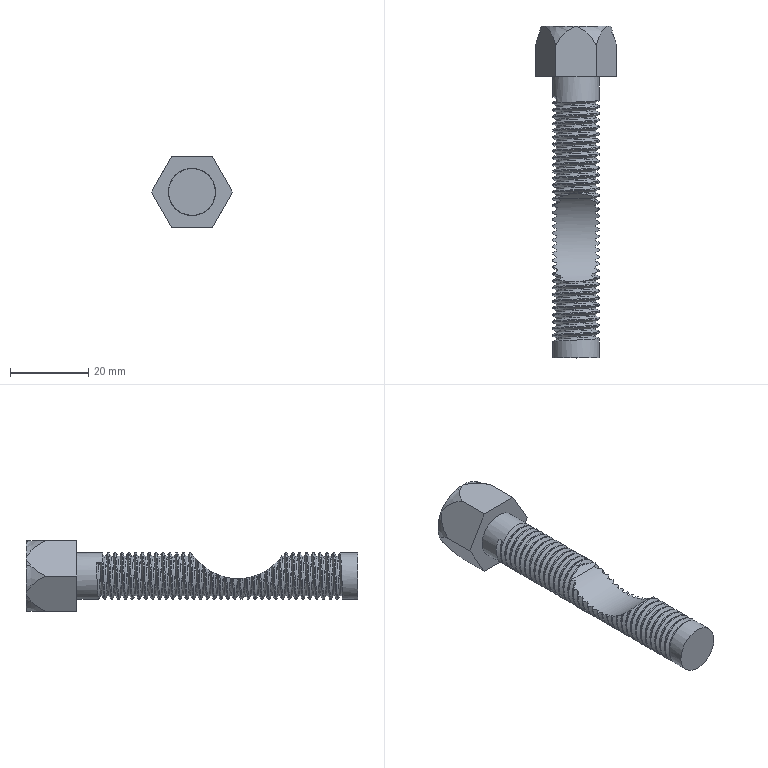Component | NX | SCREW_4 | 1 solid | 100 faces | volume 9948 mm3 | cylinder 53 | spline 28 | plane 13 | other 6 | commonest cylinder face diameters 12 x37 10.25 x13 30 x2 27.504 x1